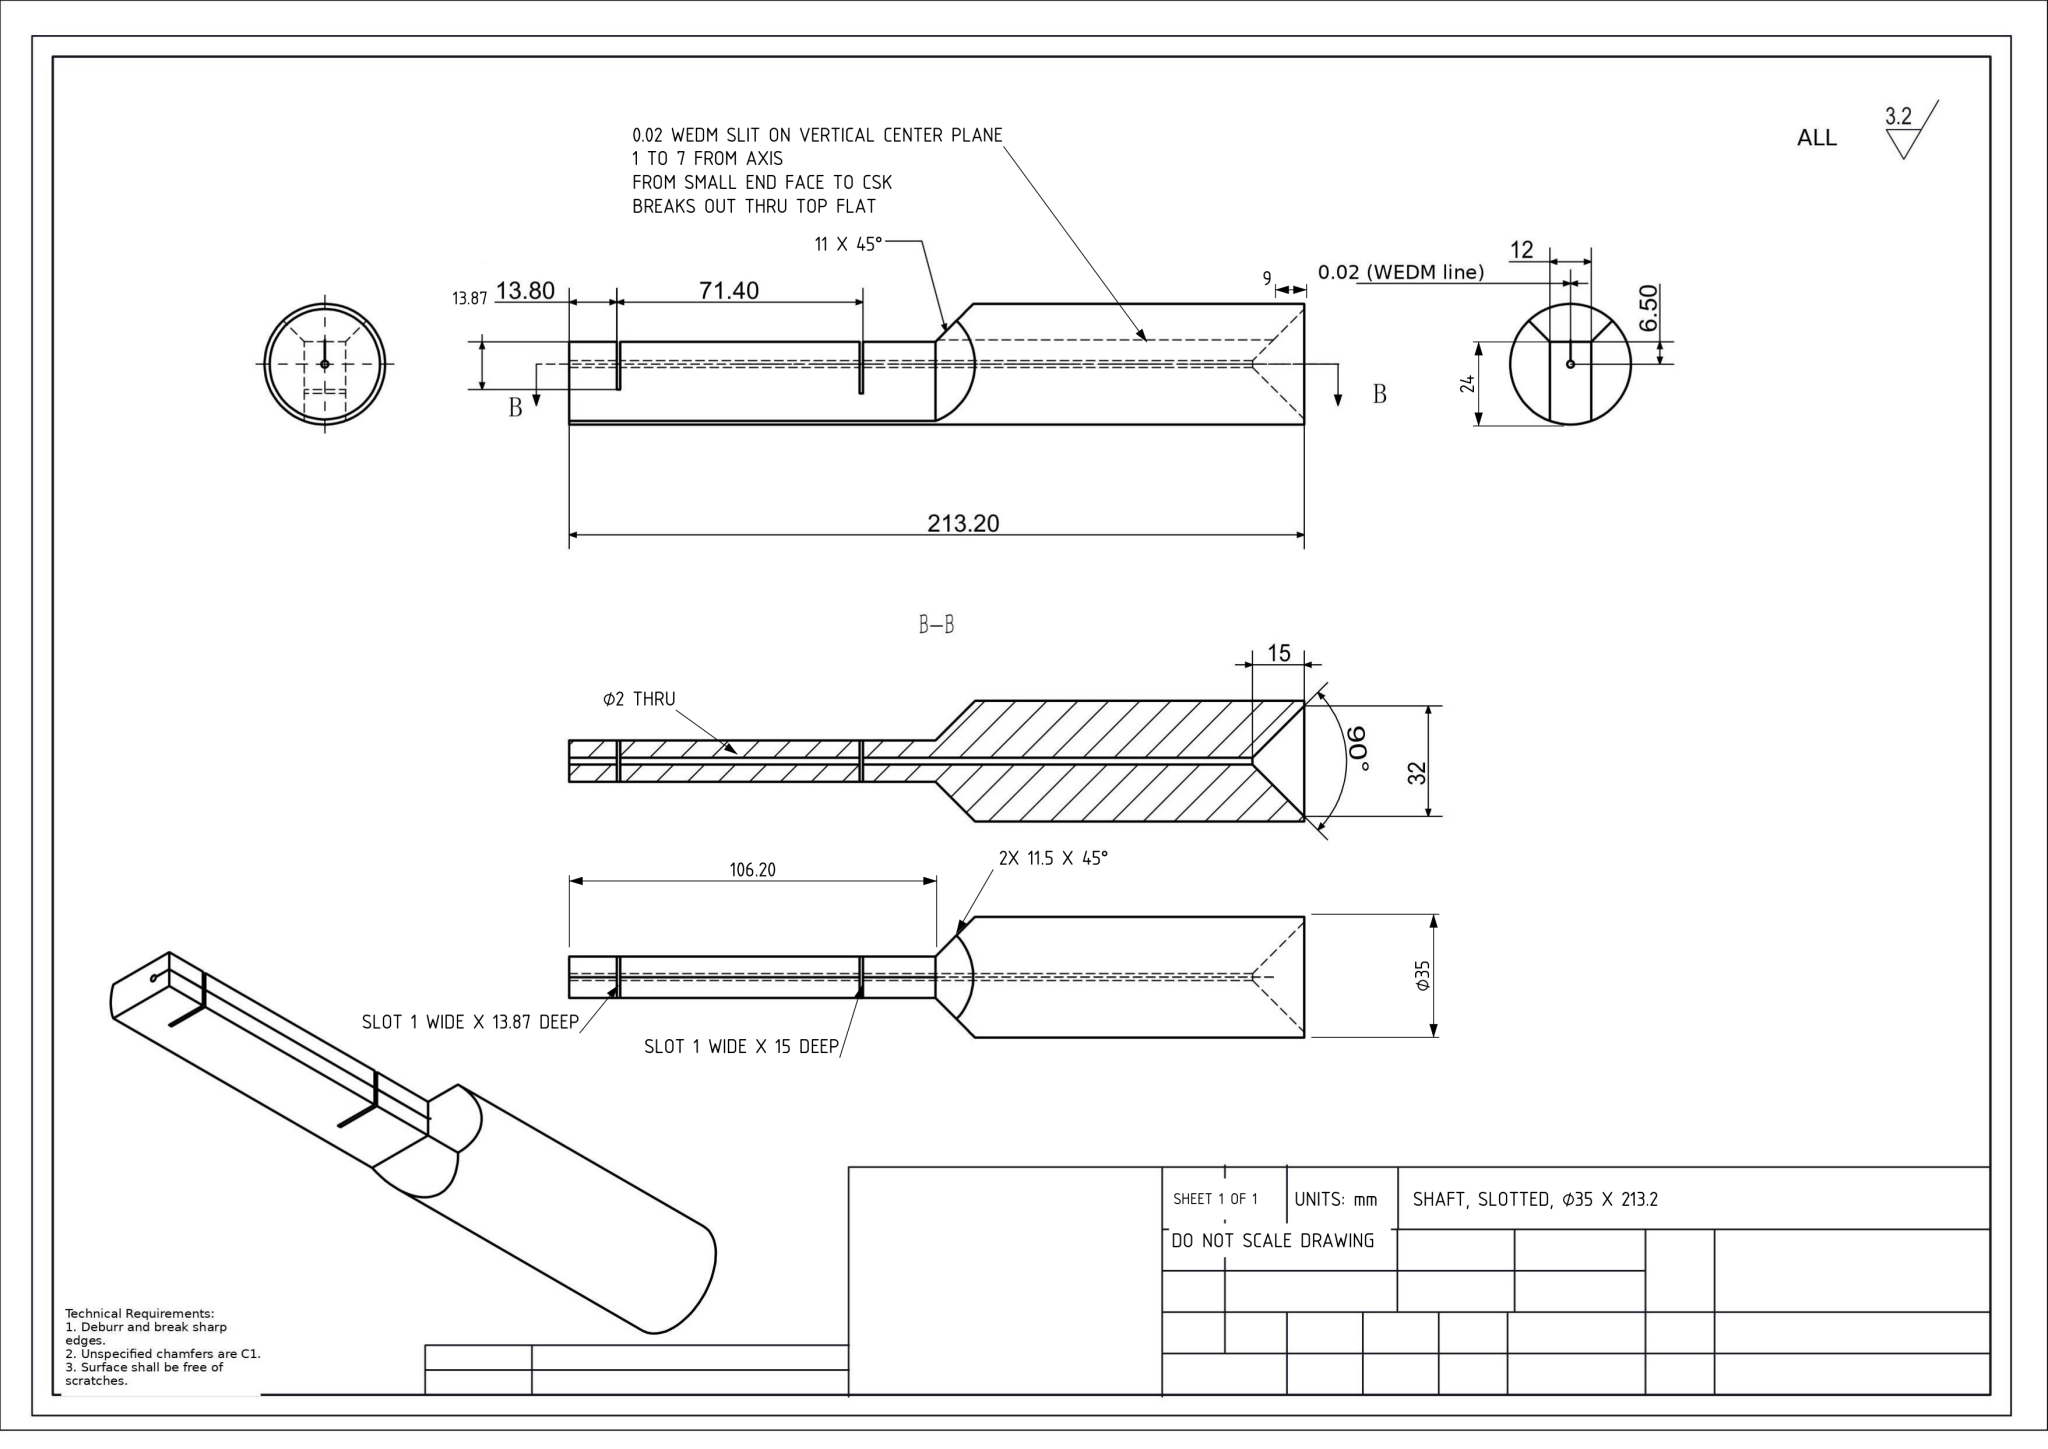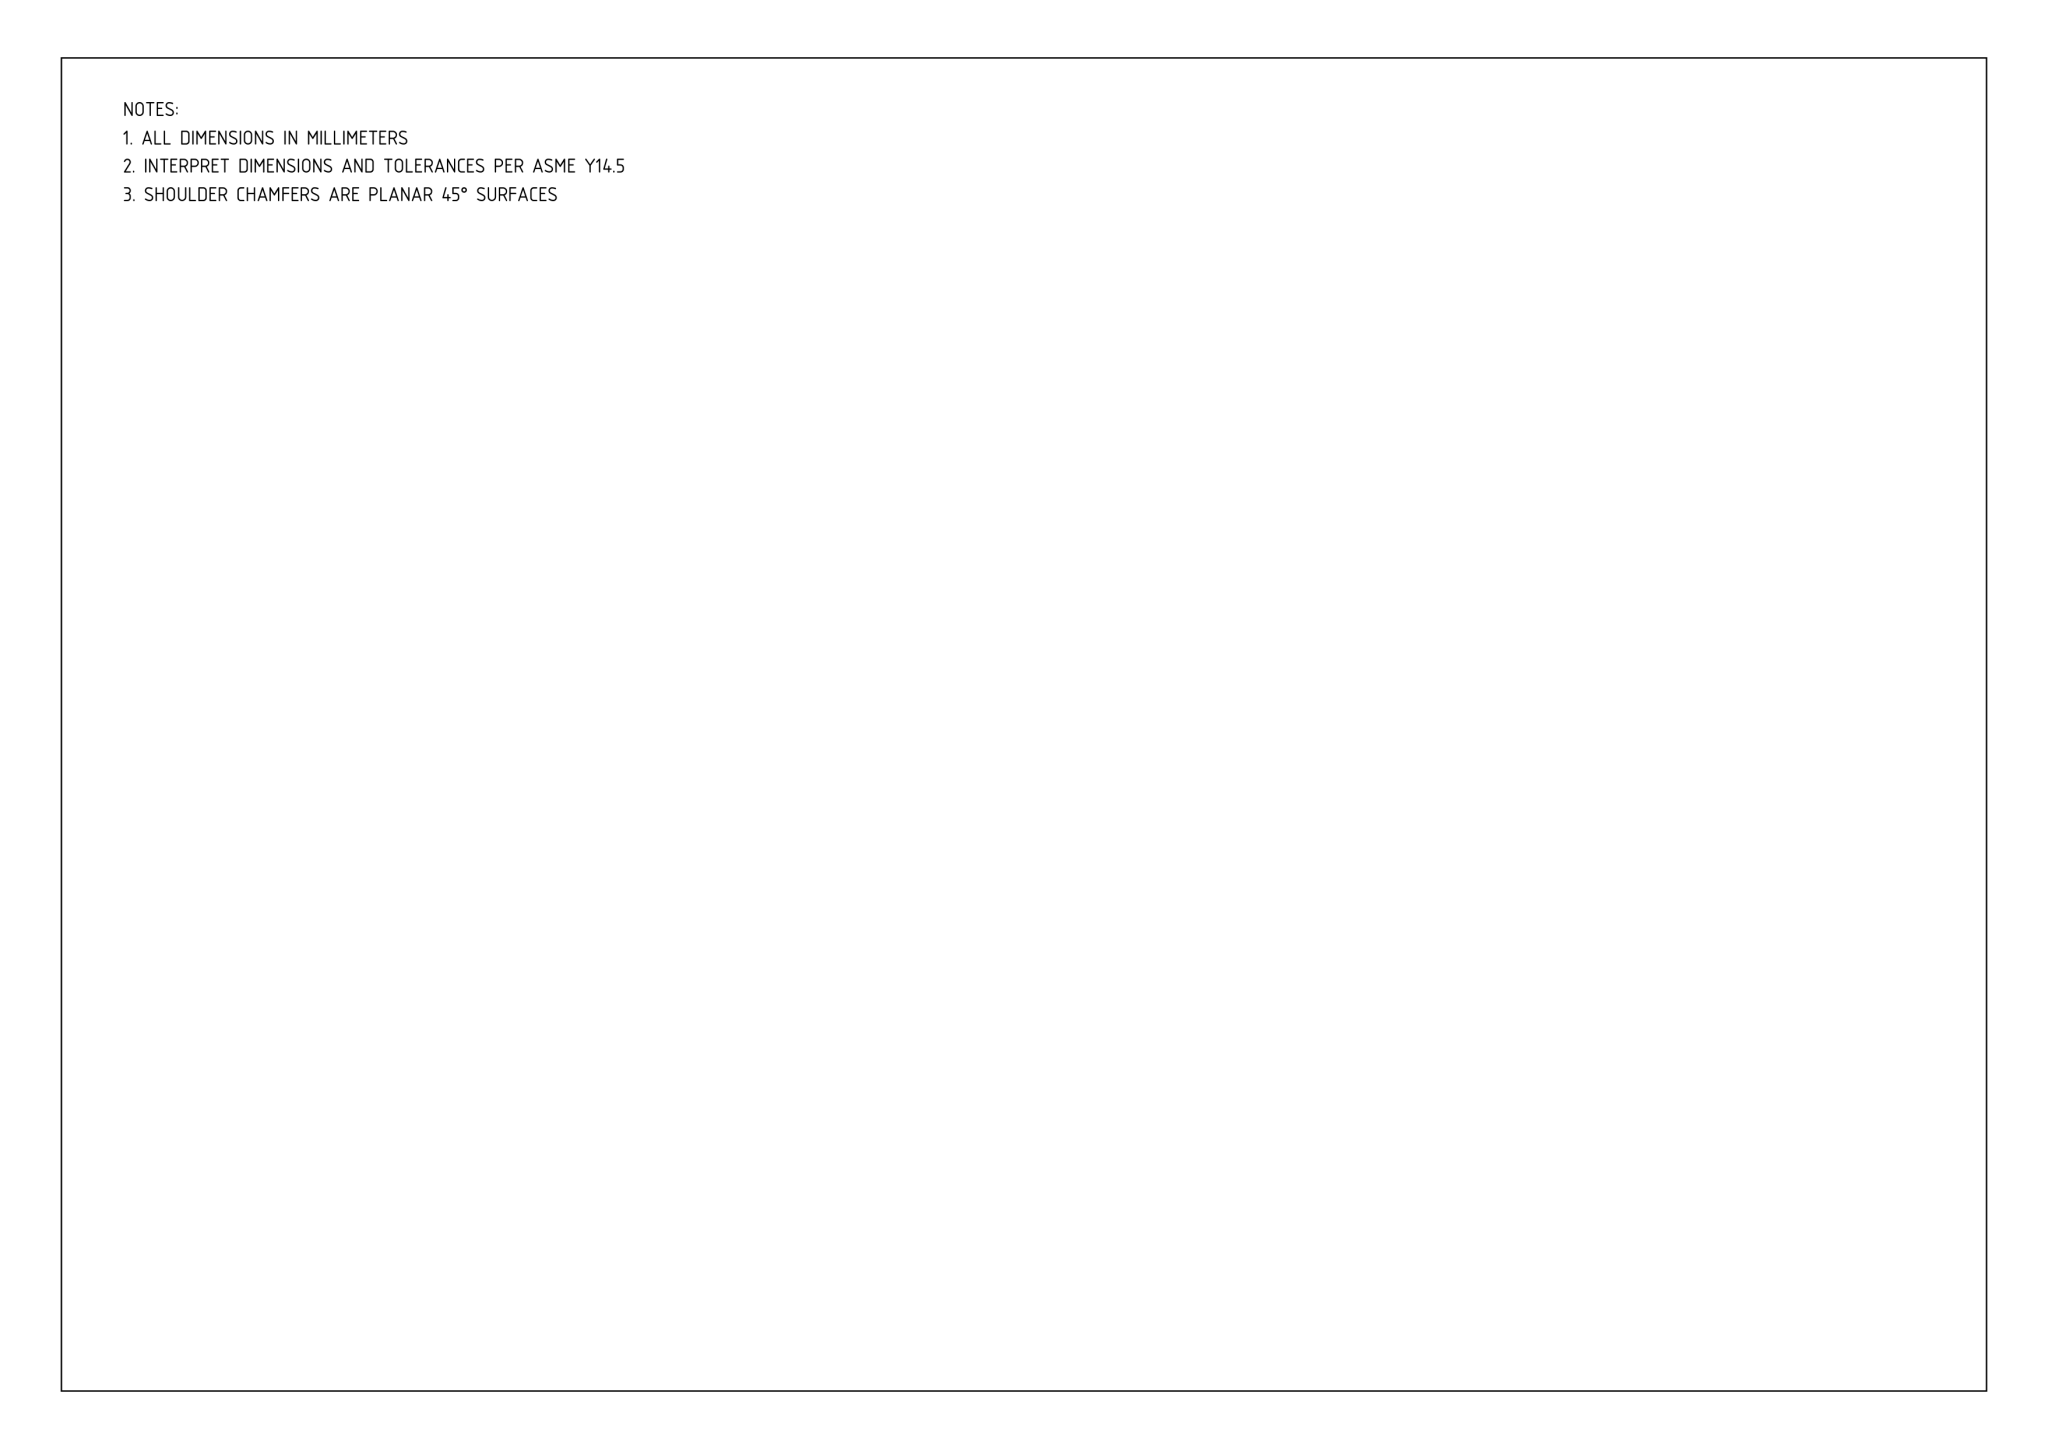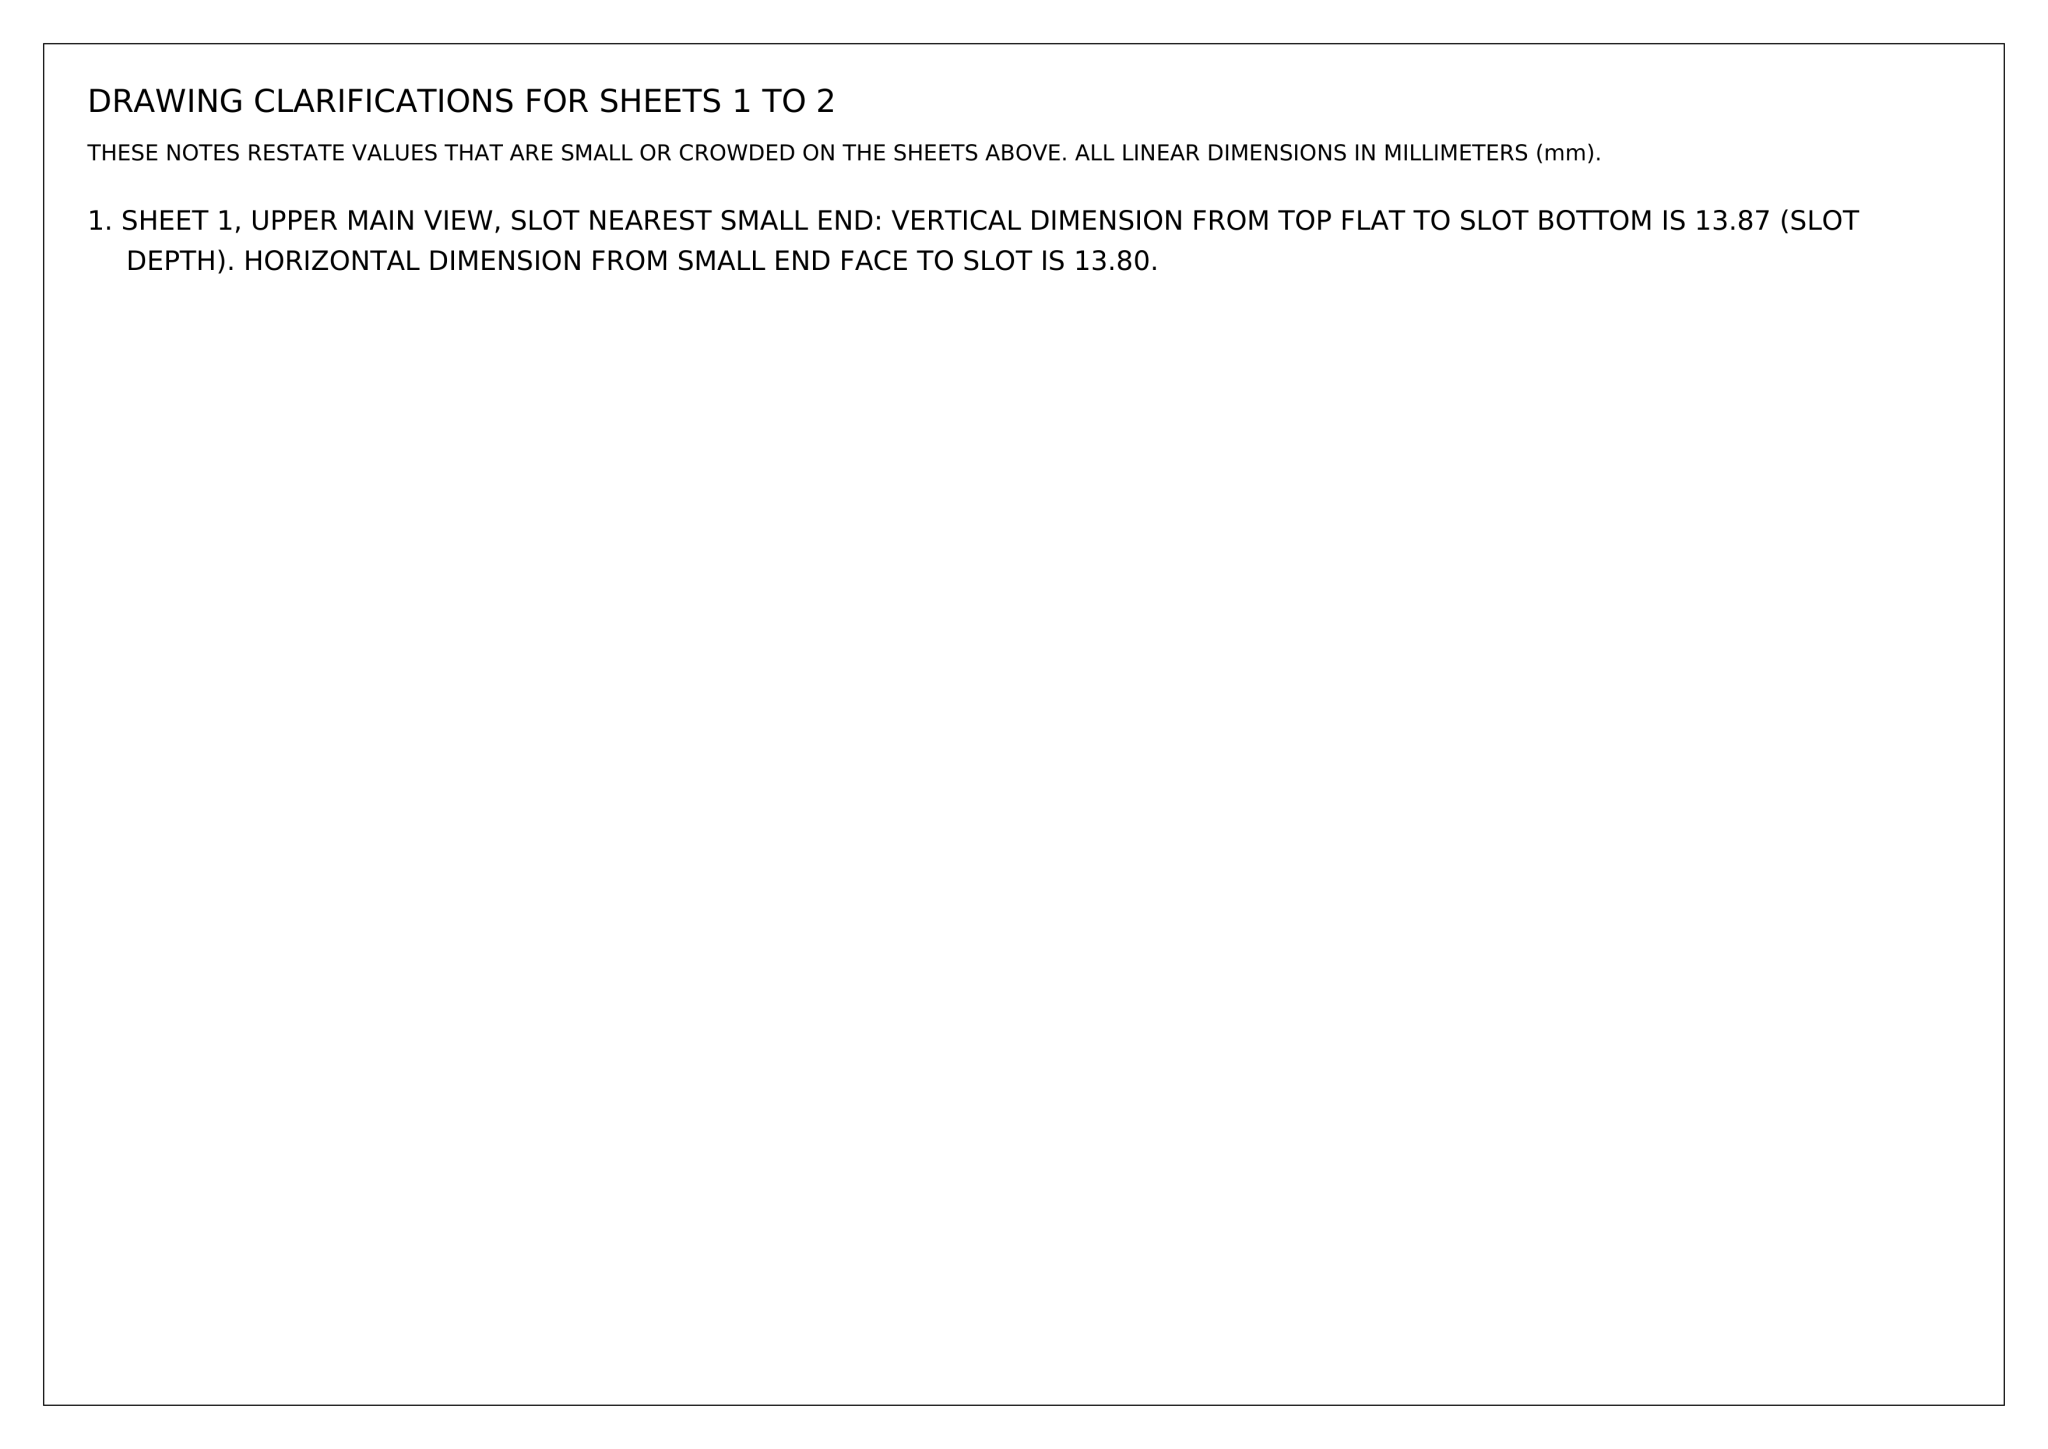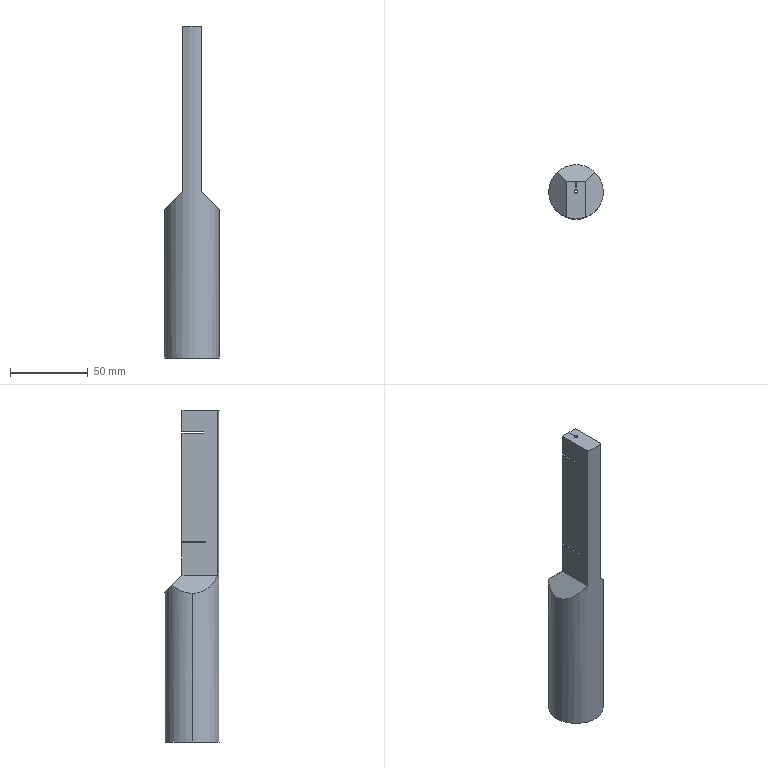Part | NX | mm | 1 solid | 39 faces | box 35 x 35 x 213.2 mm | volume 124291 mm3 | plane 26 | cylinder 11 | cone 2 | commonest cylinder face diameters 2 x9 35 x2